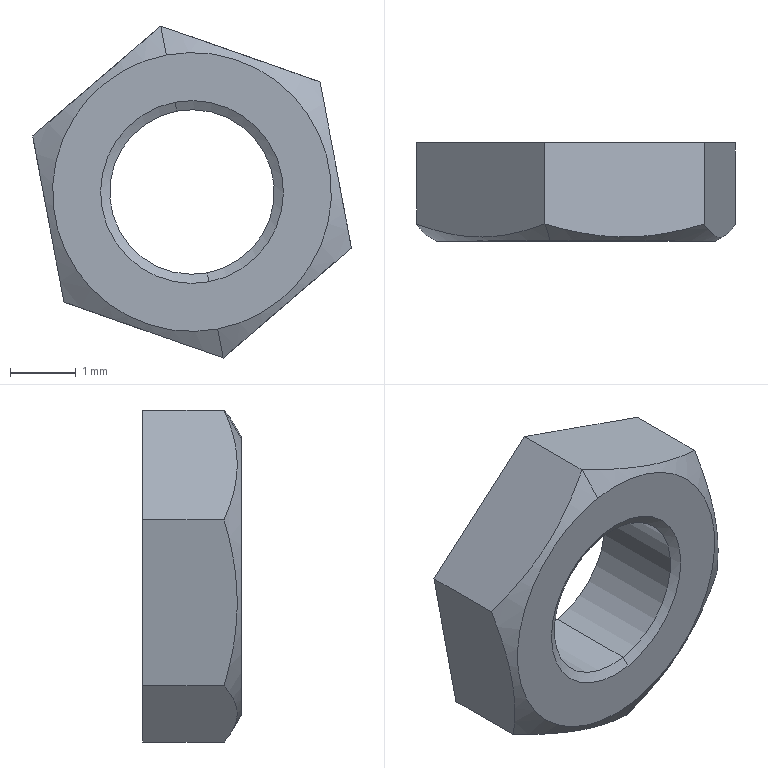Component | SolidWorks | hex nuts, style 1-grades ab gb1-12 | 1 solid | 14 faces | box 4.84 x 1.49 x 5.04 mm | volume 18 mm3 | plane 8 | cone 4 | cylinder 2 | commonest cylinder face diameters 2.5 x2
STEP:
#1=COLOUR_RGB('',0.7922,0.8196,0.9333);
#2=FILL_AREA_STYLE_COLOUR('',#1);
#3=FILL_AREA_STYLE('',(#2));
#4=SURFACE_STYLE_FILL_AREA(#3);
#5=SURFACE_SIDE_STYLE('',(#4));
#6=SURFACE_STYLE_USAGE(.BOTH.,#5);
#7=PRESENTATION_STYLE_ASSIGNMENT((#6));
#8=CARTESIAN_POINT('',(-0.6903,0.7367,2.078));
#9=VERTEX_POINT('',#8);
#10=CARTESIAN_POINT('',(-0.7085,0.7367,2.174));
#11=VERTEX_POINT('',#10);
#12=CARTESIAN_POINT('',(-0.6994,0.7367,2.126));
#13=DIRECTION('',(-0.,-1.,-0.));
#14=DIRECTION('',(-0.1846,0.,0.9828));
#15=AXIS2_PLACEMENT_3D('',#12,#13,#14);
#16=CIRCLE('',#15,0.04921);
#17=EDGE_CURVE('',#9,#11,#16,.T.);
#18=ORIENTED_EDGE('',*,*,#17,.F.);
#19=CARTESIAN_POINT('',(-0.6893,0.7335,2.072));
#20=VERTEX_POINT('',#19);
#21=CARTESIAN_POINT('',(-0.6903,0.7367,2.078));
#22=DIRECTION('',(0.1598,-0.5,-0.8511));
#23=VECTOR('',#22,39.37);
#24=LINE('',#21,#23);
#25=EDGE_CURVE('',#9,#20,#24,.T.);
#26=ORIENTED_EDGE('',*,*,#25,.T.);
#27=CARTESIAN_POINT('',(-0.7095,0.7335,2.18));
#28=VERTEX_POINT('',#27);
#29=CARTESIAN_POINT('',(-0.6994,0.7335,2.126));
#30=DIRECTION('',(0.,1.,0.));
#31=DIRECTION('',(-0.1846,0.,0.9828));
#32=AXIS2_PLACEMENT_3D('',#29,#30,#31);
#33=CIRCLE('',#32,0.05468);
#34=EDGE_CURVE('',#28,#20,#33,.T.);
#35=ORIENTED_EDGE('',*,*,#34,.F.);
#36=CARTESIAN_POINT('',(-0.7085,0.7367,2.174));
#37=DIRECTION('',(-0.1598,-0.5,0.8511));
#38=VECTOR('',#37,39.37);
#39=LINE('',#36,#38);
#40=EDGE_CURVE('',#11,#28,#39,.T.);
#41=ORIENTED_EDGE('',*,*,#40,.F.);
#42=EDGE_LOOP('',(#18,#26,#35,#41));
#43=FACE_OUTER_BOUND('',#42,.T.);
#44=CARTESIAN_POINT('',(-0.6994,0.7367,2.126));
#45=DIRECTION('',(-0.,-1.,-0.));
#46=DIRECTION('',(-0.1846,0.,0.9828));
#47=AXIS2_PLACEMENT_3D('',#44,#45,#46);
#48=CONICAL_SURFACE('',#47,0.04921,1.047);
#49=ADVANCED_FACE('',(#43),#48,.F.);
#50=CARTESIAN_POINT('',(-0.684,0.7335,2.044));
#51=VERTEX_POINT('',#50);
#52=CARTESIAN_POINT('',(-0.7148,0.7335,2.208));
#53=VERTEX_POINT('',#52);
#54=CARTESIAN_POINT('',(-0.6994,0.7335,2.126));
#55=DIRECTION('',(0.,1.,0.));
#56=DIRECTION('',(0.1846,0.,-0.9828));
#57=AXIS2_PLACEMENT_3D('',#54,#55,#56);
#58=CIRCLE('',#57,0.08339);
#59=EDGE_CURVE('',#51,#53,#58,.T.);
#60=ORIENTED_EDGE('',*,*,#59,.T.);
#61=CARTESIAN_POINT('',(-0.7181,0.7437,2.225));
#62=VERTEX_POINT('',#61);
#63=CARTESIAN_POINT('',(-0.7148,0.7335,2.208));
#64=DIRECTION('',(-0.1598,0.5,0.8511));
#65=VECTOR('',#64,39.37);
#66=LINE('',#63,#65);
#67=EDGE_CURVE('',#53,#62,#66,.T.);
#68=ORIENTED_EDGE('',*,*,#67,.T.);
#69=CARTESIAN_POINT('',(-0.7947,0.7437,2.159));
#70=VERTEX_POINT('',#69);
#71=CARTESIAN_POINT('',(-0.7181,0.7437,2.225));
#72=CARTESIAN_POINT('',(-0.7306,0.7389,2.215));
#73=CARTESIAN_POINT('',(-0.7433,0.7359,2.204));
#74=CARTESIAN_POINT('',(-0.7628,0.7359,2.187));
#75=CARTESIAN_POINT('',(-0.7694,0.7366,2.181));
#76=CARTESIAN_POINT('',(-0.7821,0.7393,2.17));
#77=CARTESIAN_POINT('',(-0.7885,0.7413,2.165));
#78=CARTESIAN_POINT('',(-0.7947,0.7437,2.159));
#79=B_SPLINE_CURVE_WITH_KNOTS('',3,(#71,#72,#73,#74,#75,#76,#77,#78),.UNSPECIFIED.,.F.,.F.,(4,2,2,4),(0.00000007,0.001296,0.001944,0.002592),.UNSPECIFIED.);
#80=EDGE_CURVE('',#62,#70,#79,.T.);
#81=ORIENTED_EDGE('',*,*,#80,.T.);
#82=CARTESIAN_POINT('',(-0.7761,0.7437,2.06));
#83=VERTEX_POINT('',#82);
#84=CARTESIAN_POINT('',(-0.7947,0.7437,2.159));
#85=CARTESIAN_POINT('',(-0.7932,0.7413,2.151));
#86=CARTESIAN_POINT('',(-0.7917,0.7394,2.143));
#87=CARTESIAN_POINT('',(-0.7886,0.7366,2.127));
#88=CARTESIAN_POINT('',(-0.787,0.7359,2.118));
#89=CARTESIAN_POINT('',(-0.7838,0.7359,2.101));
#90=CARTESIAN_POINT('',(-0.7823,0.7366,2.093));
#91=CARTESIAN_POINT('',(-0.7792,0.7393,2.077));
#92=CARTESIAN_POINT('',(-0.7776,0.7413,2.068));
#93=CARTESIAN_POINT('',(-0.7761,0.7437,2.06));
#94=B_SPLINE_CURVE_WITH_KNOTS('',3,(#84,#85,#86,#87,#88,#89,#90,#91,#92,#93),.UNSPECIFIED.,.F.,.F.,(4,2,2,2,4),(0.0009504,0.001598,0.002245,0.002893,0.00354),.UNSPECIFIED.);
#95=EDGE_CURVE('',#70,#83,#94,.T.);
#96=ORIENTED_EDGE('',*,*,#95,.T.);
#97=CARTESIAN_POINT('',(-0.6808,0.7437,2.027));
#98=VERTEX_POINT('',#97);
#99=CARTESIAN_POINT('',(-0.7761,0.7437,2.06));
#100=CARTESIAN_POINT('',(-0.7605,0.7389,2.055));
#101=CARTESIAN_POINT('',(-0.7447,0.7359,2.049));
#102=CARTESIAN_POINT('',(-0.7204,0.7359,2.041));
#103=CARTESIAN_POINT('',(-0.7123,0.7366,2.038));
#104=CARTESIAN_POINT('',(-0.6964,0.7393,2.032));
#105=CARTESIAN_POINT('',(-0.6886,0.7413,2.029));
#106=CARTESIAN_POINT('',(-0.6808,0.7437,2.027));
#107=B_SPLINE_CURVE_WITH_KNOTS('',3,(#99,#100,#101,#102,#103,#104,#105,#106),.UNSPECIFIED.,.F.,.F.,(4,2,2,4),(0.00000007,0.001296,0.001944,0.002592),.UNSPECIFIED.);
#108=EDGE_CURVE('',#83,#98,#107,.T.);
#109=ORIENTED_EDGE('',*,*,#108,.T.);
#110=CARTESIAN_POINT('',(-0.684,0.7335,2.044));
#111=DIRECTION('',(0.1598,0.5,-0.8511));
#112=VECTOR('',#111,39.37);
#113=LINE('',#110,#112);
#114=EDGE_CURVE('',#51,#98,#113,.T.);
#115=ORIENTED_EDGE('',*,*,#114,.F.);
#116=EDGE_LOOP('',(#60,#68,#81,#96,#109,#115));
#117=FACE_OUTER_BOUND('',#116,.T.);
#118=CARTESIAN_POINT('',(-0.6994,0.7335,2.126));
#119=DIRECTION('',(0.,1.,0.));
#120=DIRECTION('',(0.1846,0.,-0.9828));
#121=AXIS2_PLACEMENT_3D('',#118,#119,#120);
#122=CONICAL_SURFACE('',#121,0.08339,1.047);
#123=ADVANCED_FACE('',(#117),#122,.T.);
#124=CARTESIAN_POINT('',(-0.7085,0.7923,2.174));
#125=VERTEX_POINT('',#124);
#126=CARTESIAN_POINT('',(-0.6903,0.7923,2.078));
#127=VERTEX_POINT('',#126);
#128=CARTESIAN_POINT('',(-0.6994,0.7923,2.126));
#129=DIRECTION('',(0.,1.,0.));
#130=DIRECTION('',(-0.1846,0.,0.9828));
#131=AXIS2_PLACEMENT_3D('',#128,#129,#130);
#132=CIRCLE('',#131,0.04921);
#133=EDGE_CURVE('',#125,#127,#132,.T.);
#134=ORIENTED_EDGE('',*,*,#133,.T.);
#135=CARTESIAN_POINT('',(-0.6903,0.8254,2.078));
#136=DIRECTION('',(-0.,-1.,-0.));
#137=VECTOR('',#136,39.37);
#138=LINE('',#135,#137);
#139=EDGE_CURVE('',#127,#9,#138,.T.);
#140=ORIENTED_EDGE('',*,*,#139,.T.);
#141=ORIENTED_EDGE('',*,*,#17,.T.);
#142=CARTESIAN_POINT('',(-0.7085,0.8254,2.174));
#143=DIRECTION('',(-0.,-1.,-0.));
#144=VECTOR('',#143,39.37);
#145=LINE('',#142,#144);
#146=EDGE_CURVE('',#125,#11,#145,.T.);
#147=ORIENTED_EDGE('',*,*,#146,.F.);
#148=EDGE_LOOP('',(#134,#140,#141,#147));
#149=FACE_OUTER_BOUND('',#148,.T.);
#150=CARTESIAN_POINT('',(-0.6994,0.8254,2.126));
#151=DIRECTION('',(-0.,-1.,-0.));
#152=DIRECTION('',(-0.1846,0.,0.9828));
#153=AXIS2_PLACEMENT_3D('',#150,#151,#152);
#154=CYLINDRICAL_SURFACE('',#153,0.04921);
#155=ADVANCED_FACE('',(#149),#154,.F.);
#156=CARTESIAN_POINT('',(-0.7181,0.7923,2.225));
#157=VERTEX_POINT('',#156);
#158=CARTESIAN_POINT('',(-0.6228,0.7923,2.192));
#159=VERTEX_POINT('',#158);
#160=CARTESIAN_POINT('',(-0.6228,0.7923,2.192));
#161=DIRECTION('',(0.9434,-0.,-0.3316));
#162=VECTOR('',#161,39.37);
#163=LINE('',#160,#162);
#164=EDGE_CURVE('',#157,#159,#163,.T.);
#165=ORIENTED_EDGE('',*,*,#164,.F.);
#166=CARTESIAN_POINT('',(-0.7181,0.8254,2.225));
#167=DIRECTION('',(-0.,-1.,-0.));
#168=VECTOR('',#167,39.37);
#169=LINE('',#166,#168);
#170=EDGE_CURVE('',#157,#62,#169,.T.);
#171=ORIENTED_EDGE('',*,*,#170,.T.);
#172=CARTESIAN_POINT('',(-0.6228,0.7437,2.192));
#173=VERTEX_POINT('',#172);
#174=CARTESIAN_POINT('',(-0.6228,0.7437,2.192));
#175=CARTESIAN_POINT('',(-0.6383,0.7389,2.197));
#176=CARTESIAN_POINT('',(-0.6541,0.7359,2.203));
#177=CARTESIAN_POINT('',(-0.6784,0.7359,2.211));
#178=CARTESIAN_POINT('',(-0.6865,0.7366,2.214));
#179=CARTESIAN_POINT('',(-0.7024,0.7393,2.22));
#180=CARTESIAN_POINT('',(-0.7103,0.7413,2.223));
#181=CARTESIAN_POINT('',(-0.7181,0.7437,2.225));
#182=B_SPLINE_CURVE_WITH_KNOTS('',3,(#174,#175,#176,#177,#178,#179,#180,#181),.UNSPECIFIED.,.F.,.F.,(4,2,2,4),(0.00000007,0.001296,0.001944,0.002592),.UNSPECIFIED.);
#183=EDGE_CURVE('',#173,#62,#182,.T.);
#184=ORIENTED_EDGE('',*,*,#183,.F.);
#185=CARTESIAN_POINT('',(-0.6228,0.8254,2.192));
#186=DIRECTION('',(-0.,-1.,-0.));
#187=VECTOR('',#186,39.37);
#188=LINE('',#185,#187);
#189=EDGE_CURVE('',#159,#173,#188,.T.);
#190=ORIENTED_EDGE('',*,*,#189,.F.);
#191=EDGE_LOOP('',(#165,#171,#184,#190));
#192=FACE_OUTER_BOUND('',#191,.T.);
#193=CARTESIAN_POINT('',(-0.6228,0.8254,2.192));
#194=DIRECTION('',(0.3316,0.,0.9434));
#195=DIRECTION('',(-0.9434,0.,0.3316));
#196=AXIS2_PLACEMENT_3D('',#193,#194,#195);
#197=PLANE('',#196);
#198=ADVANCED_FACE('',(#192),#197,.T.);
#199=CARTESIAN_POINT('',(-0.6041,0.7923,2.092));
#200=VERTEX_POINT('',#199);
#201=CARTESIAN_POINT('',(-0.6041,0.7923,2.092));
#202=DIRECTION('',(0.1846,-0.,-0.9828));
#203=VECTOR('',#202,39.37);
#204=LINE('',#201,#203);
#205=EDGE_CURVE('',#159,#200,#204,.T.);
#206=ORIENTED_EDGE('',*,*,#205,.F.);
#207=ORIENTED_EDGE('',*,*,#189,.T.);
#208=CARTESIAN_POINT('',(-0.6041,0.7437,2.092));
#209=VERTEX_POINT('',#208);
#210=CARTESIAN_POINT('',(-0.6041,0.7437,2.092));
#211=CARTESIAN_POINT('',(-0.6056,0.7413,2.101));
#212=CARTESIAN_POINT('',(-0.6072,0.7393,2.109));
#213=CARTESIAN_POINT('',(-0.6103,0.7366,2.125));
#214=CARTESIAN_POINT('',(-0.6119,0.7359,2.134));
#215=CARTESIAN_POINT('',(-0.615,0.7359,2.151));
#216=CARTESIAN_POINT('',(-0.6166,0.7366,2.159));
#217=CARTESIAN_POINT('',(-0.6197,0.7394,2.176));
#218=CARTESIAN_POINT('',(-0.6212,0.7413,2.184));
#219=CARTESIAN_POINT('',(-0.6228,0.7437,2.192));
#220=B_SPLINE_CURVE_WITH_KNOTS('',3,(#210,#211,#212,#213,#214,#215,#216,#217,#218,#219),.UNSPECIFIED.,.F.,.F.,(4,2,2,2,4),(0.00228,0.002929,0.003578,0.004227,0.004876),.UNSPECIFIED.);
#221=EDGE_CURVE('',#209,#173,#220,.T.);
#222=ORIENTED_EDGE('',*,*,#221,.F.);
#223=CARTESIAN_POINT('',(-0.6041,0.8254,2.092));
#224=DIRECTION('',(-0.,-1.,-0.));
#225=VECTOR('',#224,39.37);
#226=LINE('',#223,#225);
#227=EDGE_CURVE('',#200,#209,#226,.T.);
#228=ORIENTED_EDGE('',*,*,#227,.F.);
#229=EDGE_LOOP('',(#206,#207,#222,#228));
#230=FACE_OUTER_BOUND('',#229,.T.);
#231=CARTESIAN_POINT('',(-0.6041,0.8254,2.092));
#232=DIRECTION('',(0.9828,-0.,0.1846));
#233=DIRECTION('',(0.,1.,0.));
#234=AXIS2_PLACEMENT_3D('',#231,#232,#233);
#235=PLANE('',#234);
#236=ADVANCED_FACE('',(#230),#235,.T.);
#237=CARTESIAN_POINT('',(-0.6808,0.7923,2.027));
#238=VERTEX_POINT('',#237);
#239=CARTESIAN_POINT('',(-0.6808,0.7923,2.027));
#240=DIRECTION('',(-0.7589,0.,-0.6512));
#241=VECTOR('',#240,39.37);
#242=LINE('',#239,#241);
#243=EDGE_CURVE('',#200,#238,#242,.T.);
#244=ORIENTED_EDGE('',*,*,#243,.F.);
#245=ORIENTED_EDGE('',*,*,#227,.T.);
#246=CARTESIAN_POINT('',(-0.6808,0.7437,2.027));
#247=CARTESIAN_POINT('',(-0.6683,0.7389,2.037));
#248=CARTESIAN_POINT('',(-0.6556,0.7359,2.048));
#249=CARTESIAN_POINT('',(-0.636,0.7359,2.065));
#250=CARTESIAN_POINT('',(-0.6295,0.7366,2.071));
#251=CARTESIAN_POINT('',(-0.6167,0.7393,2.082));
#252=CARTESIAN_POINT('',(-0.6104,0.7413,2.087));
#253=CARTESIAN_POINT('',(-0.6041,0.7437,2.092));
#254=B_SPLINE_CURVE_WITH_KNOTS('',3,(#246,#247,#248,#249,#250,#251,#252,#253),.UNSPECIFIED.,.F.,.F.,(4,2,2,4),(0.00000007,0.001296,0.001944,0.002592),.UNSPECIFIED.);
#255=EDGE_CURVE('',#98,#209,#254,.T.);
#256=ORIENTED_EDGE('',*,*,#255,.F.);
#257=CARTESIAN_POINT('',(-0.6808,0.8254,2.027));
#258=DIRECTION('',(-0.,-1.,-0.));
#259=VECTOR('',#258,39.37);
#260=LINE('',#257,#259);
#261=EDGE_CURVE('',#238,#98,#260,.T.);
#262=ORIENTED_EDGE('',*,*,#261,.F.);
#263=EDGE_LOOP('',(#244,#245,#256,#262));
#264=FACE_OUTER_BOUND('',#263,.T.);
#265=CARTESIAN_POINT('',(-0.6808,0.8254,2.027));
#266=DIRECTION('',(0.6512,-0.,-0.7589));
#267=DIRECTION('',(0.7589,-0.,0.6512));
#268=AXIS2_PLACEMENT_3D('',#265,#266,#267);
#269=PLANE('',#268);
#270=ADVANCED_FACE('',(#264),#269,.T.);
#271=CARTESIAN_POINT('',(-0.7761,0.7923,2.06));
#272=VERTEX_POINT('',#271);
#273=CARTESIAN_POINT('',(-0.7761,0.7923,2.06));
#274=DIRECTION('',(-0.9434,0.,0.3316));
#275=VECTOR('',#274,39.37);
#276=LINE('',#273,#275);
#277=EDGE_CURVE('',#238,#272,#276,.T.);
#278=ORIENTED_EDGE('',*,*,#277,.F.);
#279=ORIENTED_EDGE('',*,*,#261,.T.);
#280=ORIENTED_EDGE('',*,*,#108,.F.);
#281=CARTESIAN_POINT('',(-0.7761,0.8254,2.06));
#282=DIRECTION('',(-0.,-1.,-0.));
#283=VECTOR('',#282,39.37);
#284=LINE('',#281,#283);
#285=EDGE_CURVE('',#272,#83,#284,.T.);
#286=ORIENTED_EDGE('',*,*,#285,.F.);
#287=EDGE_LOOP('',(#278,#279,#280,#286));
#288=FACE_OUTER_BOUND('',#287,.T.);
#289=CARTESIAN_POINT('',(-0.7761,0.8254,2.06));
#290=DIRECTION('',(-0.3316,-0.,-0.9434));
#291=DIRECTION('',(0.9434,-0.,-0.3316));
#292=AXIS2_PLACEMENT_3D('',#289,#290,#291);
#293=PLANE('',#292);
#294=ADVANCED_FACE('',(#288),#293,.T.);
#295=CARTESIAN_POINT('',(-0.7947,0.7923,2.159));
#296=VERTEX_POINT('',#295);
#297=CARTESIAN_POINT('',(-0.7947,0.7923,2.159));
#298=DIRECTION('',(-0.1846,0.,0.9828));
#299=VECTOR('',#298,39.37);
#300=LINE('',#297,#299);
#301=EDGE_CURVE('',#272,#296,#300,.T.);
#302=ORIENTED_EDGE('',*,*,#301,.F.);
#303=ORIENTED_EDGE('',*,*,#285,.T.);
#304=ORIENTED_EDGE('',*,*,#95,.F.);
#305=CARTESIAN_POINT('',(-0.7947,0.8254,2.159));
#306=DIRECTION('',(-0.,-1.,-0.));
#307=VECTOR('',#306,39.37);
#308=LINE('',#305,#307);
#309=EDGE_CURVE('',#296,#70,#308,.T.);
#310=ORIENTED_EDGE('',*,*,#309,.F.);
#311=EDGE_LOOP('',(#302,#303,#304,#310));
#312=FACE_OUTER_BOUND('',#311,.T.);
#313=CARTESIAN_POINT('',(-0.7947,0.8254,2.159));
#314=DIRECTION('',(-0.9828,0.,-0.1846));
#315=DIRECTION('',(-0.,-1.,-0.));
#316=AXIS2_PLACEMENT_3D('',#313,#314,#315);
#317=PLANE('',#316);
#318=ADVANCED_FACE('',(#312),#317,.T.);
#319=CARTESIAN_POINT('',(-0.7181,0.7923,2.225));
#320=DIRECTION('',(0.7589,-0.,0.6512));
#321=VECTOR('',#320,39.37);
#322=LINE('',#319,#321);
#323=EDGE_CURVE('',#296,#157,#322,.T.);
#324=ORIENTED_EDGE('',*,*,#323,.F.);
#325=ORIENTED_EDGE('',*,*,#309,.T.);
#326=ORIENTED_EDGE('',*,*,#80,.F.);
#327=ORIENTED_EDGE('',*,*,#170,.F.);
#328=EDGE_LOOP('',(#324,#325,#326,#327));
#329=FACE_OUTER_BOUND('',#328,.T.);
#330=CARTESIAN_POINT('',(-0.7181,0.8254,2.225));
#331=DIRECTION('',(-0.6512,0.,0.7589));
#332=DIRECTION('',(-0.7589,0.,-0.6512));
#333=AXIS2_PLACEMENT_3D('',#330,#331,#332);
#334=PLANE('',#333);
#335=ADVANCED_FACE('',(#329),#334,.T.);
#336=ORIENTED_EDGE('',*,*,#34,.T.);
#337=CARTESIAN_POINT('',(-0.6994,0.7335,2.126));
#338=DIRECTION('',(0.,1.,0.));
#339=DIRECTION('',(-0.1846,0.,0.9828));
#340=AXIS2_PLACEMENT_3D('',#337,#338,#339);
#341=CIRCLE('',#340,0.05468);
#342=EDGE_CURVE('',#20,#28,#341,.T.);
#343=ORIENTED_EDGE('',*,*,#342,.T.);
#344=EDGE_LOOP('',(#336,#343));
#345=FACE_BOUND('',#344,.T.);
#346=ORIENTED_EDGE('',*,*,#59,.F.);
#347=CARTESIAN_POINT('',(-0.6994,0.7335,2.126));
#348=DIRECTION('',(0.,1.,0.));
#349=DIRECTION('',(0.1846,0.,-0.9828));
#350=AXIS2_PLACEMENT_3D('',#347,#348,#349);
#351=CIRCLE('',#350,0.08339);
#352=EDGE_CURVE('',#53,#51,#351,.T.);
#353=ORIENTED_EDGE('',*,*,#352,.F.);
#354=EDGE_LOOP('',(#346,#353));
#355=FACE_OUTER_BOUND('',#354,.T.);
#356=CARTESIAN_POINT('',(-0.7181,0.7335,2.225));
#357=DIRECTION('',(-0.,-1.,0.));
#358=DIRECTION('',(-0.1846,0.,0.9828));
#359=AXIS2_PLACEMENT_3D('',#356,#357,#358);
#360=PLANE('',#359);
#361=ADVANCED_FACE('',(#345,#355),#360,.T.);
#362=ORIENTED_EDGE('',*,*,#139,.F.);
#363=CARTESIAN_POINT('',(-0.6994,0.7923,2.126));
#364=DIRECTION('',(0.,1.,0.));
#365=DIRECTION('',(-0.1846,0.,0.9828));
#366=AXIS2_PLACEMENT_3D('',#363,#364,#365);
#367=CIRCLE('',#366,0.04921);
#368=EDGE_CURVE('',#127,#125,#367,.T.);
#369=ORIENTED_EDGE('',*,*,#368,.T.);
#370=ORIENTED_EDGE('',*,*,#146,.T.);
#371=CARTESIAN_POINT('',(-0.6994,0.7367,2.126));
#372=DIRECTION('',(-0.,-1.,-0.));
#373=DIRECTION('',(-0.1846,0.,0.9828));
#374=AXIS2_PLACEMENT_3D('',#371,#372,#373);
#375=CIRCLE('',#374,0.04921);
#376=EDGE_CURVE('',#11,#9,#375,.T.);
#377=ORIENTED_EDGE('',*,*,#376,.T.);
#378=EDGE_LOOP('',(#362,#369,#370,#377));
#379=FACE_OUTER_BOUND('',#378,.T.);
#380=CARTESIAN_POINT('',(-0.6994,0.8254,2.126));
#381=DIRECTION('',(-0.,-1.,-0.));
#382=DIRECTION('',(-0.1846,0.,0.9828));
#383=AXIS2_PLACEMENT_3D('',#380,#381,#382);
#384=CYLINDRICAL_SURFACE('',#383,0.04921);
#385=ADVANCED_FACE('',(#379),#384,.F.);
#386=ORIENTED_EDGE('',*,*,#67,.F.);
#387=ORIENTED_EDGE('',*,*,#352,.T.);
#388=ORIENTED_EDGE('',*,*,#114,.T.);
#389=ORIENTED_EDGE('',*,*,#255,.T.);
#390=ORIENTED_EDGE('',*,*,#221,.T.);
#391=ORIENTED_EDGE('',*,*,#183,.T.);
#392=EDGE_LOOP('',(#386,#387,#388,#389,#390,#391));
#393=FACE_OUTER_BOUND('',#392,.T.);
#394=CARTESIAN_POINT('',(-0.6994,0.7335,2.126));
#395=DIRECTION('',(0.,1.,0.));
#396=DIRECTION('',(0.1846,0.,-0.9828));
#397=AXIS2_PLACEMENT_3D('',#394,#395,#396);
#398=CONICAL_SURFACE('',#397,0.08339,1.047);
#399=ADVANCED_FACE('',(#393),#398,.T.);
#400=ORIENTED_EDGE('',*,*,#25,.F.);
#401=ORIENTED_EDGE('',*,*,#376,.F.);
#402=ORIENTED_EDGE('',*,*,#40,.T.);
#403=ORIENTED_EDGE('',*,*,#342,.F.);
#404=EDGE_LOOP('',(#400,#401,#402,#403));
#405=FACE_OUTER_BOUND('',#404,.T.);
#406=CARTESIAN_POINT('',(-0.6994,0.7367,2.126));
#407=DIRECTION('',(-0.,-1.,-0.));
#408=DIRECTION('',(-0.1846,0.,0.9828));
#409=AXIS2_PLACEMENT_3D('',#406,#407,#408);
#410=CONICAL_SURFACE('',#409,0.04921,1.047);
#411=ADVANCED_FACE('',(#405),#410,.F.);
#412=ORIENTED_EDGE('',*,*,#164,.T.);
#413=ORIENTED_EDGE('',*,*,#205,.T.);
#414=ORIENTED_EDGE('',*,*,#243,.T.);
#415=ORIENTED_EDGE('',*,*,#277,.T.);
#416=ORIENTED_EDGE('',*,*,#301,.T.);
#417=ORIENTED_EDGE('',*,*,#323,.T.);
#418=EDGE_LOOP('',(#412,#413,#414,#415,#416,#417));
#419=FACE_OUTER_BOUND('',#418,.T.);
#420=ORIENTED_EDGE('',*,*,#133,.F.);
#421=ORIENTED_EDGE('',*,*,#368,.F.);
#422=EDGE_LOOP('',(#420,#421));
#423=FACE_BOUND('',#422,.T.);
#424=CARTESIAN_POINT('',(-0.6994,0.7923,2.126));
#425=DIRECTION('',(-0.,-1.,0.));
#426=DIRECTION('',(-0.1846,0.,0.9828));
#427=AXIS2_PLACEMENT_3D('',#424,#425,#426);
#428=PLANE('',#427);
#429=ADVANCED_FACE('',(#419,#423),#428,.F.);
#430=CLOSED_SHELL('',(#49,#123,#155,#198,#236,#270,#294,#318,#335,#361,#385,#399,#411,#429));
#431=MANIFOLD_SOLID_BREP('',#430);
#432=STYLED_ITEM('',(#7),#431);
#433=(LENGTH_UNIT()NAMED_UNIT(*)SI_UNIT($,.METRE.));
#434=LENGTH_MEASURE_WITH_UNIT(LENGTH_MEASURE(0.0254),#433);
#435=DIMENSIONAL_EXPONENTS(1.,0.,0.,0.,0.,0.,0.);
#436=(CONVERSION_BASED_UNIT('',#434)LENGTH_UNIT()NAMED_UNIT(#435));
#437=UNCERTAINTY_MEASURE_WITH_UNIT(LENGTH_MEASURE(0.00001),#436,'','');
#438=(NAMED_UNIT(*)PLANE_ANGLE_UNIT()SI_UNIT($,.RADIAN.));
#439=(NAMED_UNIT(*)SI_UNIT($,.STERADIAN.)SOLID_ANGLE_UNIT());
#440=(GEOMETRIC_REPRESENTATION_CONTEXT(3)GLOBAL_UNCERTAINTY_ASSIGNED_CONTEXT((#437))GLOBAL_UNIT_ASSIGNED_CONTEXT((#436,#438,#439))REPRESENTATION_CONTEXT('',''));
#441=MECHANICAL_DESIGN_GEOMETRIC_PRESENTATION_REPRESENTATION('',(#432),#440);
#442=PRESENTATION_LAYER_ASSIGNMENT('','',(#432));
#443=CARTESIAN_POINT('',(0.,0.,0.));
#444=DIRECTION('',(0.,0.,1.));
#445=DIRECTION('',(1.,0.,0.));
#446=AXIS2_PLACEMENT_3D('',#443,#444,#445);
#447=(LENGTH_UNIT()NAMED_UNIT(*)SI_UNIT($,.METRE.));
#448=LENGTH_MEASURE_WITH_UNIT(LENGTH_MEASURE(0.0254),#447);
#449=DIMENSIONAL_EXPONENTS(1.,0.,0.,0.,0.,0.,0.);
#450=(CONVERSION_BASED_UNIT('',#448)LENGTH_UNIT()NAMED_UNIT(#449));
#451=UNCERTAINTY_MEASURE_WITH_UNIT(LENGTH_MEASURE(0.00001),#450,'','');
#452=(NAMED_UNIT(*)PLANE_ANGLE_UNIT()SI_UNIT($,.RADIAN.));
#453=(NAMED_UNIT(*)SI_UNIT($,.STERADIAN.)SOLID_ANGLE_UNIT());
#454=(GEOMETRIC_REPRESENTATION_CONTEXT(3)GLOBAL_UNCERTAINTY_ASSIGNED_CONTEXT((#451))GLOBAL_UNIT_ASSIGNED_CONTEXT((#450,#452,#453))REPRESENTATION_CONTEXT('',''));
#455=ADVANCED_BREP_SHAPE_REPRESENTATION('',(#431,#446),#454);